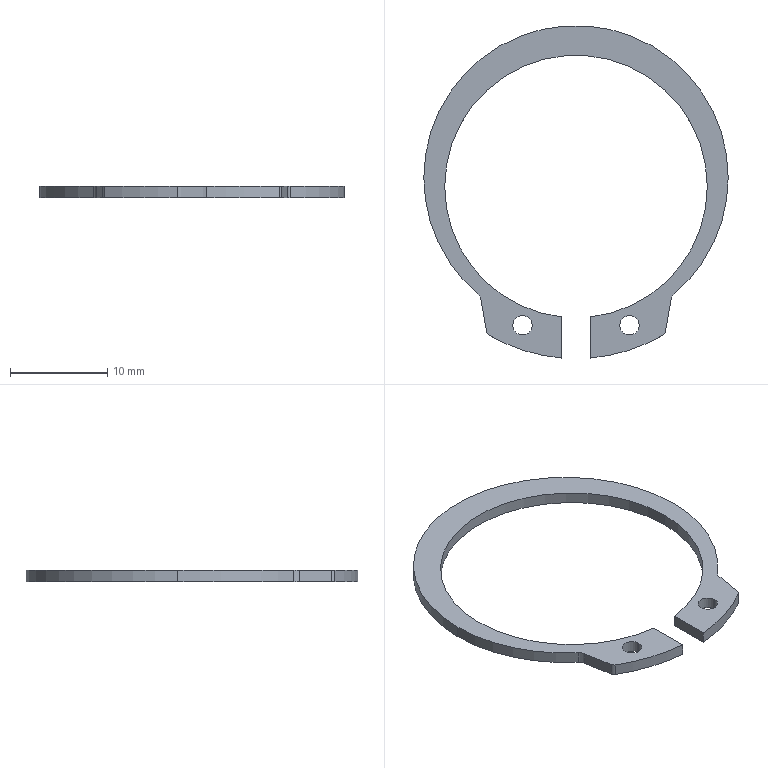Component | SolidWorks | 28mmShaftSnapRingGB896-1986-28-1 | 1 solid | 22 faces | box 31.3 x 34.19 x 1.2 mm | volume 284 mm3 | cylinder 16 | plane 6 | commonest cylinder face diameters 2 x6 31.3 x3 27 x3 1 x2 35.4 x2
STEP:
#1=CARTESIAN_POINT('',(-18.936,-4.841,97.87));
#2=VERTEX_POINT('',#1);
#3=CARTESIAN_POINT('',(-20.168,-4.841,97.87));
#4=VERTEX_POINT('',#3);
#5=CARTESIAN_POINT('',(-19.552,-4.841,97.87));
#6=DIRECTION('',(0.,0.,1.));
#7=DIRECTION('',(1.,0.,0.));
#8=AXIS2_PLACEMENT_3D('',#5,#6,#7);
#9=CIRCLE('',#8,0.6161);
#10=EDGE_CURVE('',#2,#4,#9,.T.);
#11=ORIENTED_EDGE('',*,*,#10,.T.);
#12=CARTESIAN_POINT('',(-20.168,-4.841,97.917));
#13=VERTEX_POINT('',#12);
#14=CARTESIAN_POINT('',(-20.168,-4.841,97.87));
#15=DIRECTION('',(0.,0.,1.));
#16=VECTOR('',#15,39.37);
#17=LINE('',#14,#16);
#18=EDGE_CURVE('',#4,#13,#17,.T.);
#19=ORIENTED_EDGE('',*,*,#18,.T.);
#20=CARTESIAN_POINT('',(-18.936,-4.841,97.917));
#21=VERTEX_POINT('',#20);
#22=CARTESIAN_POINT('',(-19.552,-4.841,97.917));
#23=DIRECTION('',(0.,0.,-1.));
#24=DIRECTION('',(1.,0.,0.));
#25=AXIS2_PLACEMENT_3D('',#22,#23,#24);
#26=CIRCLE('',#25,0.6161);
#27=EDGE_CURVE('',#13,#21,#26,.T.);
#28=ORIENTED_EDGE('',*,*,#27,.T.);
#29=CARTESIAN_POINT('',(-18.936,-4.841,97.87));
#30=DIRECTION('',(0.,0.,1.));
#31=VECTOR('',#30,39.37);
#32=LINE('',#29,#31);
#33=EDGE_CURVE('',#2,#21,#32,.T.);
#34=ORIENTED_EDGE('',*,*,#33,.F.);
#35=EDGE_LOOP('',(#11,#19,#28,#34));
#36=FACE_OUTER_BOUND('',#35,.T.);
#37=CARTESIAN_POINT('',(-19.552,-4.841,97.87));
#38=DIRECTION('',(0.,0.,1.));
#39=DIRECTION('',(1.,0.,0.));
#40=AXIS2_PLACEMENT_3D('',#37,#38,#39);
#41=CYLINDRICAL_SURFACE('',#40,0.6161);
#42=ADVANCED_FACE('',(#36),#41,.T.);
#43=CARTESIAN_POINT('',(-19.153,-5.312,97.87));
#44=VERTEX_POINT('',#43);
#45=CARTESIAN_POINT('',(-19.552,-4.841,97.87));
#46=DIRECTION('',(0.,0.,1.));
#47=DIRECTION('',(1.,0.,0.));
#48=AXIS2_PLACEMENT_3D('',#45,#46,#47);
#49=CIRCLE('',#48,0.6161);
#50=EDGE_CURVE('',#44,#2,#49,.T.);
#51=ORIENTED_EDGE('',*,*,#50,.T.);
#52=ORIENTED_EDGE('',*,*,#33,.T.);
#53=CARTESIAN_POINT('',(-19.153,-5.312,97.917));
#54=VERTEX_POINT('',#53);
#55=CARTESIAN_POINT('',(-19.552,-4.841,97.917));
#56=DIRECTION('',(0.,0.,-1.));
#57=DIRECTION('',(1.,0.,0.));
#58=AXIS2_PLACEMENT_3D('',#55,#56,#57);
#59=CIRCLE('',#58,0.6161);
#60=EDGE_CURVE('',#21,#54,#59,.T.);
#61=ORIENTED_EDGE('',*,*,#60,.T.);
#62=CARTESIAN_POINT('',(-19.153,-5.312,97.87));
#63=DIRECTION('',(0.,0.,-1.));
#64=VECTOR('',#63,39.37);
#65=LINE('',#62,#64);
#66=EDGE_CURVE('',#54,#44,#65,.T.);
#67=ORIENTED_EDGE('',*,*,#66,.T.);
#68=EDGE_LOOP('',(#51,#52,#61,#67));
#69=FACE_OUTER_BOUND('',#68,.T.);
#70=CARTESIAN_POINT('',(-19.552,-4.841,97.87));
#71=DIRECTION('',(0.,0.,1.));
#72=DIRECTION('',(1.,0.,0.));
#73=AXIS2_PLACEMENT_3D('',#70,#71,#72);
#74=CYLINDRICAL_SURFACE('',#73,0.6161);
#75=ADVANCED_FACE('',(#69),#74,.T.);
#76=CARTESIAN_POINT('',(-20.083,-4.877,97.87));
#77=VERTEX_POINT('',#76);
#78=CARTESIAN_POINT('',(-19.611,-5.405,97.87));
#79=VERTEX_POINT('',#78);
#80=CARTESIAN_POINT('',(-19.552,-4.877,97.87));
#81=DIRECTION('',(0.,0.,1.));
#82=DIRECTION('',(-1.,0.,0.));
#83=AXIS2_PLACEMENT_3D('',#80,#81,#82);
#84=CIRCLE('',#83,0.5315);
#85=EDGE_CURVE('',#77,#79,#84,.T.);
#86=ORIENTED_EDGE('',*,*,#85,.F.);
#87=CARTESIAN_POINT('',(-20.083,-4.877,97.917));
#88=VERTEX_POINT('',#87);
#89=CARTESIAN_POINT('',(-20.083,-4.877,97.87));
#90=DIRECTION('',(0.,0.,1.));
#91=VECTOR('',#90,39.37);
#92=LINE('',#89,#91);
#93=EDGE_CURVE('',#77,#88,#92,.T.);
#94=ORIENTED_EDGE('',*,*,#93,.T.);
#95=CARTESIAN_POINT('',(-19.611,-5.405,97.917));
#96=VERTEX_POINT('',#95);
#97=CARTESIAN_POINT('',(-19.552,-4.877,97.917));
#98=DIRECTION('',(0.,0.,1.));
#99=DIRECTION('',(-1.,0.,0.));
#100=AXIS2_PLACEMENT_3D('',#97,#98,#99);
#101=CIRCLE('',#100,0.5315);
#102=EDGE_CURVE('',#88,#96,#101,.T.);
#103=ORIENTED_EDGE('',*,*,#102,.T.);
#104=CARTESIAN_POINT('',(-19.611,-5.405,97.87));
#105=DIRECTION('',(0.,0.,1.));
#106=VECTOR('',#105,39.37);
#107=LINE('',#104,#106);
#108=EDGE_CURVE('',#79,#96,#107,.T.);
#109=ORIENTED_EDGE('',*,*,#108,.F.);
#110=EDGE_LOOP('',(#86,#94,#103,#109));
#111=FACE_OUTER_BOUND('',#110,.T.);
#112=CARTESIAN_POINT('',(-19.552,-4.877,97.87));
#113=DIRECTION('',(0.,0.,1.));
#114=DIRECTION('',(1.,0.,0.));
#115=AXIS2_PLACEMENT_3D('',#112,#113,#114);
#116=CYLINDRICAL_SURFACE('',#115,0.5315);
#117=ADVANCED_FACE('',(#111),#116,.F.);
#118=ORIENTED_EDGE('',*,*,#93,.F.);
#119=CARTESIAN_POINT('',(-19.02,-4.877,97.87));
#120=VERTEX_POINT('',#119);
#121=CARTESIAN_POINT('',(-19.552,-4.877,97.87));
#122=DIRECTION('',(0.,0.,1.));
#123=DIRECTION('',(-1.,0.,0.));
#124=AXIS2_PLACEMENT_3D('',#121,#122,#123);
#125=CIRCLE('',#124,0.5315);
#126=EDGE_CURVE('',#120,#77,#125,.T.);
#127=ORIENTED_EDGE('',*,*,#126,.F.);
#128=CARTESIAN_POINT('',(-19.02,-4.877,97.917));
#129=VERTEX_POINT('',#128);
#130=CARTESIAN_POINT('',(-19.02,-4.877,97.87));
#131=DIRECTION('',(0.,0.,1.));
#132=VECTOR('',#131,39.37);
#133=LINE('',#130,#132);
#134=EDGE_CURVE('',#120,#129,#133,.T.);
#135=ORIENTED_EDGE('',*,*,#134,.T.);
#136=CARTESIAN_POINT('',(-19.552,-4.877,97.917));
#137=DIRECTION('',(0.,0.,1.));
#138=DIRECTION('',(-1.,0.,0.));
#139=AXIS2_PLACEMENT_3D('',#136,#137,#138);
#140=CIRCLE('',#139,0.5315);
#141=EDGE_CURVE('',#129,#88,#140,.T.);
#142=ORIENTED_EDGE('',*,*,#141,.T.);
#143=EDGE_LOOP('',(#118,#127,#135,#142));
#144=FACE_OUTER_BOUND('',#143,.T.);
#145=CARTESIAN_POINT('',(-19.552,-4.877,97.87));
#146=DIRECTION('',(0.,0.,1.));
#147=DIRECTION('',(1.,0.,0.));
#148=AXIS2_PLACEMENT_3D('',#145,#146,#147);
#149=CYLINDRICAL_SURFACE('',#148,0.5315);
#150=ADVANCED_FACE('',(#144),#149,.F.);
#151=CARTESIAN_POINT('',(-19.808,-5.439,97.87));
#152=VERTEX_POINT('',#151);
#153=CARTESIAN_POINT('',(-19.729,-5.439,97.87));
#154=VERTEX_POINT('',#153);
#155=CARTESIAN_POINT('',(-19.768,-5.439,97.87));
#156=DIRECTION('',(0.,0.,1.));
#157=DIRECTION('',(1.,0.,0.));
#158=AXIS2_PLACEMENT_3D('',#155,#156,#157);
#159=CIRCLE('',#158,0.03937);
#160=EDGE_CURVE('',#152,#154,#159,.T.);
#161=ORIENTED_EDGE('',*,*,#160,.F.);
#162=CARTESIAN_POINT('',(-19.808,-5.439,97.917));
#163=VERTEX_POINT('',#162);
#164=CARTESIAN_POINT('',(-19.808,-5.439,97.87));
#165=DIRECTION('',(0.,0.,1.));
#166=VECTOR('',#165,39.37);
#167=LINE('',#164,#166);
#168=EDGE_CURVE('',#152,#163,#167,.T.);
#169=ORIENTED_EDGE('',*,*,#168,.T.);
#170=CARTESIAN_POINT('',(-19.729,-5.439,97.917));
#171=VERTEX_POINT('',#170);
#172=CARTESIAN_POINT('',(-19.768,-5.439,97.917));
#173=DIRECTION('',(0.,0.,1.));
#174=DIRECTION('',(1.,0.,0.));
#175=AXIS2_PLACEMENT_3D('',#172,#173,#174);
#176=CIRCLE('',#175,0.03937);
#177=EDGE_CURVE('',#163,#171,#176,.T.);
#178=ORIENTED_EDGE('',*,*,#177,.T.);
#179=CARTESIAN_POINT('',(-19.729,-5.439,97.87));
#180=DIRECTION('',(0.,0.,1.));
#181=VECTOR('',#180,39.37);
#182=LINE('',#179,#181);
#183=EDGE_CURVE('',#154,#171,#182,.T.);
#184=ORIENTED_EDGE('',*,*,#183,.F.);
#185=EDGE_LOOP('',(#161,#169,#178,#184));
#186=FACE_OUTER_BOUND('',#185,.T.);
#187=CARTESIAN_POINT('',(-19.768,-5.439,97.87));
#188=DIRECTION('',(0.,0.,1.));
#189=DIRECTION('',(1.,0.,0.));
#190=AXIS2_PLACEMENT_3D('',#187,#188,#189);
#191=CYLINDRICAL_SURFACE('',#190,0.03937);
#192=ADVANCED_FACE('',(#186),#191,.F.);
#193=CARTESIAN_POINT('',(-19.374,-5.439,97.87));
#194=VERTEX_POINT('',#193);
#195=CARTESIAN_POINT('',(-19.296,-5.439,97.87));
#196=VERTEX_POINT('',#195);
#197=CARTESIAN_POINT('',(-19.335,-5.439,97.87));
#198=DIRECTION('',(0.,0.,1.));
#199=DIRECTION('',(1.,0.,0.));
#200=AXIS2_PLACEMENT_3D('',#197,#198,#199);
#201=CIRCLE('',#200,0.03937);
#202=EDGE_CURVE('',#194,#196,#201,.T.);
#203=ORIENTED_EDGE('',*,*,#202,.F.);
#204=CARTESIAN_POINT('',(-19.374,-5.439,97.917));
#205=VERTEX_POINT('',#204);
#206=CARTESIAN_POINT('',(-19.374,-5.439,97.87));
#207=DIRECTION('',(0.,0.,1.));
#208=VECTOR('',#207,39.37);
#209=LINE('',#206,#208);
#210=EDGE_CURVE('',#194,#205,#209,.T.);
#211=ORIENTED_EDGE('',*,*,#210,.T.);
#212=CARTESIAN_POINT('',(-19.296,-5.439,97.917));
#213=VERTEX_POINT('',#212);
#214=CARTESIAN_POINT('',(-19.335,-5.439,97.917));
#215=DIRECTION('',(0.,0.,1.));
#216=DIRECTION('',(1.,0.,0.));
#217=AXIS2_PLACEMENT_3D('',#214,#215,#216);
#218=CIRCLE('',#217,0.03937);
#219=EDGE_CURVE('',#205,#213,#218,.T.);
#220=ORIENTED_EDGE('',*,*,#219,.T.);
#221=CARTESIAN_POINT('',(-19.296,-5.439,97.87));
#222=DIRECTION('',(0.,0.,1.));
#223=VECTOR('',#222,39.37);
#224=LINE('',#221,#223);
#225=EDGE_CURVE('',#196,#213,#224,.T.);
#226=ORIENTED_EDGE('',*,*,#225,.F.);
#227=EDGE_LOOP('',(#203,#211,#220,#226));
#228=FACE_OUTER_BOUND('',#227,.T.);
#229=CARTESIAN_POINT('',(-19.335,-5.439,97.87));
#230=DIRECTION('',(0.,0.,1.));
#231=DIRECTION('',(1.,0.,0.));
#232=AXIS2_PLACEMENT_3D('',#229,#230,#231);
#233=CYLINDRICAL_SURFACE('',#232,0.03937);
#234=ADVANCED_FACE('',(#228),#233,.F.);
#235=CARTESIAN_POINT('',(-19.167,-5.335,97.917));
#236=VERTEX_POINT('',#235);
#237=CARTESIAN_POINT('',(-19.128,-5.342,97.917));
#238=DIRECTION('',(0.,0.,1.));
#239=DIRECTION('',(1.,0.,0.));
#240=AXIS2_PLACEMENT_3D('',#237,#238,#239);
#241=CIRCLE('',#240,0.03937);
#242=EDGE_CURVE('',#54,#236,#241,.T.);
#243=ORIENTED_EDGE('',*,*,#242,.F.);
#244=ORIENTED_EDGE('',*,*,#60,.F.);
#245=ORIENTED_EDGE('',*,*,#27,.F.);
#246=CARTESIAN_POINT('',(-19.95,-5.312,97.917));
#247=VERTEX_POINT('',#246);
#248=CARTESIAN_POINT('',(-19.552,-4.841,97.917));
#249=DIRECTION('',(0.,0.,-1.));
#250=DIRECTION('',(1.,0.,0.));
#251=AXIS2_PLACEMENT_3D('',#248,#249,#250);
#252=CIRCLE('',#251,0.6161);
#253=EDGE_CURVE('',#247,#13,#252,.T.);
#254=ORIENTED_EDGE('',*,*,#253,.F.);
#255=CARTESIAN_POINT('',(-19.937,-5.335,97.917));
#256=VERTEX_POINT('',#255);
#257=CARTESIAN_POINT('',(-19.975,-5.342,97.917));
#258=DIRECTION('',(0.,0.,1.));
#259=DIRECTION('',(1.,0.,0.));
#260=AXIS2_PLACEMENT_3D('',#257,#258,#259);
#261=CIRCLE('',#260,0.03937);
#262=EDGE_CURVE('',#256,#247,#261,.T.);
#263=ORIENTED_EDGE('',*,*,#262,.F.);
#264=CARTESIAN_POINT('',(-19.914,-5.464,97.917));
#265=VERTEX_POINT('',#264);
#266=CARTESIAN_POINT('',(-19.914,-5.464,97.917));
#267=DIRECTION('',(-0.1736,0.9848,0.));
#268=VECTOR('',#267,39.37);
#269=LINE('',#266,#268);
#270=EDGE_CURVE('',#265,#256,#269,.T.);
#271=ORIENTED_EDGE('',*,*,#270,.F.);
#272=CARTESIAN_POINT('',(-19.904,-5.478,97.917));
#273=VERTEX_POINT('',#272);
#274=CARTESIAN_POINT('',(-19.894,-5.461,97.917));
#275=DIRECTION('',(0.,0.,-1.));
#276=DIRECTION('',(1.,0.,0.));
#277=AXIS2_PLACEMENT_3D('',#274,#275,#276);
#278=CIRCLE('',#277,0.01969);
#279=EDGE_CURVE('',#273,#265,#278,.T.);
#280=ORIENTED_EDGE('',*,*,#279,.F.);
#281=CARTESIAN_POINT('',(-19.611,-5.571,97.917));
#282=VERTEX_POINT('',#281);
#283=CARTESIAN_POINT('',(-19.552,-4.877,97.917));
#284=DIRECTION('',(0.,0.,-1.));
#285=DIRECTION('',(1.,0.,0.));
#286=AXIS2_PLACEMENT_3D('',#283,#284,#285);
#287=CIRCLE('',#286,0.6969);
#288=EDGE_CURVE('',#282,#273,#287,.T.);
#289=ORIENTED_EDGE('',*,*,#288,.F.);
#290=CARTESIAN_POINT('',(-19.611,-4.877,97.917));
#291=DIRECTION('',(0.,-1.,0.));
#292=VECTOR('',#291,39.37);
#293=LINE('',#290,#292);
#294=EDGE_CURVE('',#96,#282,#293,.T.);
#295=ORIENTED_EDGE('',*,*,#294,.F.);
#296=ORIENTED_EDGE('',*,*,#102,.F.);
#297=ORIENTED_EDGE('',*,*,#141,.F.);
#298=CARTESIAN_POINT('',(-19.493,-5.405,97.917));
#299=VERTEX_POINT('',#298);
#300=CARTESIAN_POINT('',(-19.552,-4.877,97.917));
#301=DIRECTION('',(0.,0.,1.));
#302=DIRECTION('',(-1.,0.,0.));
#303=AXIS2_PLACEMENT_3D('',#300,#301,#302);
#304=CIRCLE('',#303,0.5315);
#305=EDGE_CURVE('',#299,#129,#304,.T.);
#306=ORIENTED_EDGE('',*,*,#305,.F.);
#307=CARTESIAN_POINT('',(-19.493,-5.571,97.917));
#308=VERTEX_POINT('',#307);
#309=CARTESIAN_POINT('',(-19.493,-4.877,97.917));
#310=DIRECTION('',(0.,1.,0.));
#311=VECTOR('',#310,39.37);
#312=LINE('',#309,#311);
#313=EDGE_CURVE('',#308,#299,#312,.T.);
#314=ORIENTED_EDGE('',*,*,#313,.F.);
#315=CARTESIAN_POINT('',(-19.199,-5.478,97.917));
#316=VERTEX_POINT('',#315);
#317=CARTESIAN_POINT('',(-19.552,-4.877,97.917));
#318=DIRECTION('',(0.,0.,-1.));
#319=DIRECTION('',(1.,0.,0.));
#320=AXIS2_PLACEMENT_3D('',#317,#318,#319);
#321=CIRCLE('',#320,0.6969);
#322=EDGE_CURVE('',#316,#308,#321,.T.);
#323=ORIENTED_EDGE('',*,*,#322,.F.);
#324=CARTESIAN_POINT('',(-19.19,-5.464,97.917));
#325=VERTEX_POINT('',#324);
#326=CARTESIAN_POINT('',(-19.209,-5.461,97.917));
#327=DIRECTION('',(0.,0.,-1.));
#328=DIRECTION('',(1.,0.,0.));
#329=AXIS2_PLACEMENT_3D('',#326,#327,#328);
#330=CIRCLE('',#329,0.01969);
#331=EDGE_CURVE('',#325,#316,#330,.T.);
#332=ORIENTED_EDGE('',*,*,#331,.F.);
#333=CARTESIAN_POINT('',(-19.167,-5.335,97.917));
#334=DIRECTION('',(-0.1736,-0.9848,0.));
#335=VECTOR('',#334,39.37);
#336=LINE('',#333,#335);
#337=EDGE_CURVE('',#236,#325,#336,.T.);
#338=ORIENTED_EDGE('',*,*,#337,.F.);
#339=EDGE_LOOP('',(#243,#244,#245,#254,#263,#271,#280,#289,#295,#296,#297,#306,#314,#323,#332,#338));
#340=FACE_OUTER_BOUND('',#339,.T.);
#341=CARTESIAN_POINT('',(-19.768,-5.439,97.917));
#342=DIRECTION('',(0.,0.,1.));
#343=DIRECTION('',(1.,0.,0.));
#344=AXIS2_PLACEMENT_3D('',#341,#342,#343);
#345=CIRCLE('',#344,0.03937);
#346=EDGE_CURVE('',#171,#163,#345,.T.);
#347=ORIENTED_EDGE('',*,*,#346,.F.);
#348=ORIENTED_EDGE('',*,*,#177,.F.);
#349=EDGE_LOOP('',(#347,#348));
#350=FACE_BOUND('',#349,.T.);
#351=CARTESIAN_POINT('',(-19.335,-5.439,97.917));
#352=DIRECTION('',(0.,0.,1.));
#353=DIRECTION('',(1.,0.,0.));
#354=AXIS2_PLACEMENT_3D('',#351,#352,#353);
#355=CIRCLE('',#354,0.03937);
#356=EDGE_CURVE('',#213,#205,#355,.T.);
#357=ORIENTED_EDGE('',*,*,#356,.F.);
#358=ORIENTED_EDGE('',*,*,#219,.F.);
#359=EDGE_LOOP('',(#357,#358));
#360=FACE_BOUND('',#359,.T.);
#361=CARTESIAN_POINT('',(-19.552,-4.877,97.917));
#362=DIRECTION('',(0.,0.,-1.));
#363=DIRECTION('',(-1.,0.,0.));
#364=AXIS2_PLACEMENT_3D('',#361,#362,#363);
#365=PLANE('',#364);
#366=ADVANCED_FACE('',(#340,#350,#360),#365,.F.);
#367=ORIENTED_EDGE('',*,*,#18,.F.);
#368=CARTESIAN_POINT('',(-19.95,-5.312,97.87));
#369=VERTEX_POINT('',#368);
#370=CARTESIAN_POINT('',(-19.552,-4.841,97.87));
#371=DIRECTION('',(0.,0.,1.));
#372=DIRECTION('',(1.,0.,0.));
#373=AXIS2_PLACEMENT_3D('',#370,#371,#372);
#374=CIRCLE('',#373,0.6161);
#375=EDGE_CURVE('',#4,#369,#374,.T.);
#376=ORIENTED_EDGE('',*,*,#375,.T.);
#377=CARTESIAN_POINT('',(-19.95,-5.312,97.87));
#378=DIRECTION('',(0.,0.,1.));
#379=VECTOR('',#378,39.37);
#380=LINE('',#377,#379);
#381=EDGE_CURVE('',#369,#247,#380,.T.);
#382=ORIENTED_EDGE('',*,*,#381,.T.);
#383=ORIENTED_EDGE('',*,*,#253,.T.);
#384=EDGE_LOOP('',(#367,#376,#382,#383));
#385=FACE_OUTER_BOUND('',#384,.T.);
#386=CARTESIAN_POINT('',(-19.552,-4.841,97.87));
#387=DIRECTION('',(0.,0.,1.));
#388=DIRECTION('',(1.,0.,0.));
#389=AXIS2_PLACEMENT_3D('',#386,#387,#388);
#390=CYLINDRICAL_SURFACE('',#389,0.6161);
#391=ADVANCED_FACE('',(#385),#390,.T.);
#392=CARTESIAN_POINT('',(-19.937,-5.335,97.87));
#393=VERTEX_POINT('',#392);
#394=CARTESIAN_POINT('',(-19.937,-5.335,97.87));
#395=DIRECTION('',(0.,0.,-1.));
#396=VECTOR('',#395,39.37);
#397=LINE('',#394,#396);
#398=EDGE_CURVE('',#256,#393,#397,.T.);
#399=ORIENTED_EDGE('',*,*,#398,.F.);
#400=ORIENTED_EDGE('',*,*,#262,.T.);
#401=ORIENTED_EDGE('',*,*,#381,.F.);
#402=CARTESIAN_POINT('',(-19.975,-5.342,97.87));
#403=DIRECTION('',(0.,0.,1.));
#404=DIRECTION('',(1.,0.,0.));
#405=AXIS2_PLACEMENT_3D('',#402,#403,#404);
#406=CIRCLE('',#405,0.03937);
#407=EDGE_CURVE('',#393,#369,#406,.T.);
#408=ORIENTED_EDGE('',*,*,#407,.F.);
#409=EDGE_LOOP('',(#399,#400,#401,#408));
#410=FACE_OUTER_BOUND('',#409,.T.);
#411=CARTESIAN_POINT('',(-19.975,-5.342,97.87));
#412=DIRECTION('',(0.,0.,1.));
#413=DIRECTION('',(1.,0.,0.));
#414=AXIS2_PLACEMENT_3D('',#411,#412,#413);
#415=CYLINDRICAL_SURFACE('',#414,0.03937);
#416=ADVANCED_FACE('',(#410),#415,.F.);
#417=CARTESIAN_POINT('',(-19.914,-5.464,97.87));
#418=VERTEX_POINT('',#417);
#419=CARTESIAN_POINT('',(-19.939,-5.321,97.87));
#420=DIRECTION('',(0.1736,-0.9848,0.));
#421=VECTOR('',#420,39.37);
#422=LINE('',#419,#421);
#423=EDGE_CURVE('',#393,#418,#422,.T.);
#424=ORIENTED_EDGE('',*,*,#423,.T.);
#425=CARTESIAN_POINT('',(-19.914,-5.464,97.87));
#426=DIRECTION('',(0.,0.,1.));
#427=VECTOR('',#426,39.37);
#428=LINE('',#425,#427);
#429=EDGE_CURVE('',#418,#265,#428,.T.);
#430=ORIENTED_EDGE('',*,*,#429,.T.);
#431=ORIENTED_EDGE('',*,*,#270,.T.);
#432=ORIENTED_EDGE('',*,*,#398,.T.);
#433=EDGE_LOOP('',(#424,#430,#431,#432));
#434=FACE_OUTER_BOUND('',#433,.T.);
#435=CARTESIAN_POINT('',(-19.939,-5.321,97.87));
#436=DIRECTION('',(-0.9848,-0.1736,0.));
#437=DIRECTION('',(0.1736,-0.9848,0.));
#438=AXIS2_PLACEMENT_3D('',#435,#436,#437);
#439=PLANE('',#438);
#440=ADVANCED_FACE('',(#434),#439,.T.);
#441=ORIENTED_EDGE('',*,*,#279,.T.);
#442=ORIENTED_EDGE('',*,*,#429,.F.);
#443=CARTESIAN_POINT('',(-19.904,-5.478,97.87));
#444=VERTEX_POINT('',#443);
#445=CARTESIAN_POINT('',(-19.894,-5.461,97.87));
#446=DIRECTION('',(0.,0.,1.));
#447=DIRECTION('',(1.,0.,0.));
#448=AXIS2_PLACEMENT_3D('',#445,#446,#447);
#449=CIRCLE('',#448,0.01969);
#450=EDGE_CURVE('',#418,#444,#449,.T.);
#451=ORIENTED_EDGE('',*,*,#450,.T.);
#452=CARTESIAN_POINT('',(-19.904,-5.478,97.87));
#453=DIRECTION('',(0.,0.,1.));
#454=VECTOR('',#453,39.37);
#455=LINE('',#452,#454);
#456=EDGE_CURVE('',#444,#273,#455,.T.);
#457=ORIENTED_EDGE('',*,*,#456,.T.);
#458=EDGE_LOOP('',(#441,#442,#451,#457));
#459=FACE_OUTER_BOUND('',#458,.T.);
#460=CARTESIAN_POINT('',(-19.894,-5.461,97.87));
#461=DIRECTION('',(0.,0.,1.));
#462=DIRECTION('',(1.,0.,0.));
#463=AXIS2_PLACEMENT_3D('',#460,#461,#462);
#464=CYLINDRICAL_SURFACE('',#463,0.01969);
#465=ADVANCED_FACE('',(#459),#464,.T.);
#466=CARTESIAN_POINT('',(-19.611,-5.571,97.87));
#467=VERTEX_POINT('',#466);
#468=CARTESIAN_POINT('',(-19.552,-4.877,97.87));
#469=DIRECTION('',(0.,0.,1.));
#470=DIRECTION('',(1.,0.,0.));
#471=AXIS2_PLACEMENT_3D('',#468,#469,#470);
#472=CIRCLE('',#471,0.6969);
#473=EDGE_CURVE('',#444,#467,#472,.T.);
#474=ORIENTED_EDGE('',*,*,#473,.T.);
#475=CARTESIAN_POINT('',(-19.611,-5.571,97.87));
#476=DIRECTION('',(0.,0.,1.));
#477=VECTOR('',#476,39.37);
#478=LINE('',#475,#477);
#479=EDGE_CURVE('',#467,#282,#478,.T.);
#480=ORIENTED_EDGE('',*,*,#479,.T.);
#481=ORIENTED_EDGE('',*,*,#288,.T.);
#482=ORIENTED_EDGE('',*,*,#456,.F.);
#483=EDGE_LOOP('',(#474,#480,#481,#482));
#484=FACE_OUTER_BOUND('',#483,.T.);
#485=CARTESIAN_POINT('',(-19.552,-4.877,97.87));
#486=DIRECTION('',(0.,0.,1.));
#487=DIRECTION('',(1.,0.,0.));
#488=AXIS2_PLACEMENT_3D('',#485,#486,#487);
#489=CYLINDRICAL_SURFACE('',#488,0.6969);
#490=ADVANCED_FACE('',(#484),#489,.T.);
#491=CARTESIAN_POINT('',(-19.611,-5.383,97.87));
#492=DIRECTION('',(0.,1.,0.));
#493=VECTOR('',#492,39.37);
#494=LINE('',#491,#493);
#495=EDGE_CURVE('',#467,#79,#494,.T.);
#496=ORIENTED_EDGE('',*,*,#495,.T.);
#497=ORIENTED_EDGE('',*,*,#108,.T.);
#498=ORIENTED_EDGE('',*,*,#294,.T.);
#499=ORIENTED_EDGE('',*,*,#479,.F.);
#500=EDGE_LOOP('',(#496,#497,#498,#499));
#501=FACE_OUTER_BOUND('',#500,.T.);
#502=CARTESIAN_POINT('',(-19.611,-5.383,97.87));
#503=DIRECTION('',(1.,0.,0.));
#504=DIRECTION('',(0.,0.,-1.));
#505=AXIS2_PLACEMENT_3D('',#502,#503,#504);
#506=PLANE('',#505);
#507=ADVANCED_FACE('',(#501),#506,.T.);
#508=ORIENTED_EDGE('',*,*,#134,.F.);
#509=CARTESIAN_POINT('',(-19.493,-5.405,97.87));
#510=VERTEX_POINT('',#509);
#511=CARTESIAN_POINT('',(-19.552,-4.877,97.87));
#512=DIRECTION('',(0.,0.,1.));
#513=DIRECTION('',(-1.,0.,0.));
#514=AXIS2_PLACEMENT_3D('',#511,#512,#513);
#515=CIRCLE('',#514,0.5315);
#516=EDGE_CURVE('',#510,#120,#515,.T.);
#517=ORIENTED_EDGE('',*,*,#516,.F.);
#518=CARTESIAN_POINT('',(-19.493,-5.405,97.917));
#519=DIRECTION('',(0.,0.,-1.));
#520=VECTOR('',#519,39.37);
#521=LINE('',#518,#520);
#522=EDGE_CURVE('',#299,#510,#521,.T.);
#523=ORIENTED_EDGE('',*,*,#522,.F.);
#524=ORIENTED_EDGE('',*,*,#305,.T.);
#525=EDGE_LOOP('',(#508,#517,#523,#524));
#526=FACE_OUTER_BOUND('',#525,.T.);
#527=CARTESIAN_POINT('',(-19.552,-4.877,97.87));
#528=DIRECTION('',(0.,0.,1.));
#529=DIRECTION('',(1.,0.,0.));
#530=AXIS2_PLACEMENT_3D('',#527,#528,#529);
#531=CYLINDRICAL_SURFACE('',#530,0.5315);
#532=ADVANCED_FACE('',(#526),#531,.F.);
#533=CARTESIAN_POINT('',(-19.493,-5.571,97.87));
#534=VERTEX_POINT('',#533);
#535=CARTESIAN_POINT('',(-19.493,-5.383,97.87));
#536=DIRECTION('',(0.,-1.,0.));
#537=VECTOR('',#536,39.37);
#538=LINE('',#535,#537);
#539=EDGE_CURVE('',#510,#534,#538,.T.);
#540=ORIENTED_EDGE('',*,*,#539,.T.);
#541=CARTESIAN_POINT('',(-19.493,-5.571,97.87));
#542=DIRECTION('',(0.,0.,1.));
#543=VECTOR('',#542,39.37);
#544=LINE('',#541,#543);
#545=EDGE_CURVE('',#534,#308,#544,.T.);
#546=ORIENTED_EDGE('',*,*,#545,.T.);
#547=ORIENTED_EDGE('',*,*,#313,.T.);
#548=ORIENTED_EDGE('',*,*,#522,.T.);
#549=EDGE_LOOP('',(#540,#546,#547,#548));
#550=FACE_OUTER_BOUND('',#549,.T.);
#551=CARTESIAN_POINT('',(-19.493,-5.383,97.87));
#552=DIRECTION('',(-1.,0.,0.));
#553=DIRECTION('',(0.,0.,1.));
#554=AXIS2_PLACEMENT_3D('',#551,#552,#553);
#555=PLANE('',#554);
#556=ADVANCED_FACE('',(#550),#555,.T.);
#557=ORIENTED_EDGE('',*,*,#322,.T.);
#558=ORIENTED_EDGE('',*,*,#545,.F.);
#559=CARTESIAN_POINT('',(-19.199,-5.478,97.87));
#560=VERTEX_POINT('',#559);
#561=CARTESIAN_POINT('',(-19.552,-4.877,97.87));
#562=DIRECTION('',(0.,0.,1.));
#563=DIRECTION('',(1.,0.,0.));
#564=AXIS2_PLACEMENT_3D('',#561,#562,#563);
#565=CIRCLE('',#564,0.6969);
#566=EDGE_CURVE('',#534,#560,#565,.T.);
#567=ORIENTED_EDGE('',*,*,#566,.T.);
#568=CARTESIAN_POINT('',(-19.199,-5.478,97.87));
#569=DIRECTION('',(0.,0.,1.));
#570=VECTOR('',#569,39.37);
#571=LINE('',#568,#570);
#572=EDGE_CURVE('',#560,#316,#571,.T.);
#573=ORIENTED_EDGE('',*,*,#572,.T.);
#574=EDGE_LOOP('',(#557,#558,#567,#573));
#575=FACE_OUTER_BOUND('',#574,.T.);
#576=CARTESIAN_POINT('',(-19.552,-4.877,97.87));
#577=DIRECTION('',(0.,0.,1.));
#578=DIRECTION('',(1.,0.,0.));
#579=AXIS2_PLACEMENT_3D('',#576,#577,#578);
#580=CYLINDRICAL_SURFACE('',#579,0.6969);
#581=ADVANCED_FACE('',(#575),#580,.T.);
#582=ORIENTED_EDGE('',*,*,#331,.T.);
#583=ORIENTED_EDGE('',*,*,#572,.F.);
#584=CARTESIAN_POINT('',(-19.19,-5.464,97.87));
#585=VERTEX_POINT('',#584);
#586=CARTESIAN_POINT('',(-19.209,-5.461,97.87));
#587=DIRECTION('',(0.,0.,1.));
#588=DIRECTION('',(1.,0.,0.));
#589=AXIS2_PLACEMENT_3D('',#586,#587,#588);
#590=CIRCLE('',#589,0.01969);
#591=EDGE_CURVE('',#560,#585,#590,.T.);
#592=ORIENTED_EDGE('',*,*,#591,.T.);
#593=CARTESIAN_POINT('',(-19.19,-5.464,97.87));
#594=DIRECTION('',(0.,0.,1.));
#595=VECTOR('',#594,39.37);
#596=LINE('',#593,#595);
#597=EDGE_CURVE('',#585,#325,#596,.T.);
#598=ORIENTED_EDGE('',*,*,#597,.T.);
#599=EDGE_LOOP('',(#582,#583,#592,#598));
#600=FACE_OUTER_BOUND('',#599,.T.);
#601=CARTESIAN_POINT('',(-19.209,-5.461,97.87));
#602=DIRECTION('',(0.,0.,1.));
#603=DIRECTION('',(1.,0.,0.));
#604=AXIS2_PLACEMENT_3D('',#601,#602,#603);
#605=CYLINDRICAL_SURFACE('',#604,0.01969);
#606=ADVANCED_FACE('',(#600),#605,.T.);
#607=ORIENTED_EDGE('',*,*,#337,.T.);
#608=ORIENTED_EDGE('',*,*,#597,.F.);
#609=CARTESIAN_POINT('',(-19.167,-5.335,97.87));
#610=VERTEX_POINT('',#609);
#611=CARTESIAN_POINT('',(-19.164,-5.321,97.87));
#612=DIRECTION('',(0.1736,0.9848,0.));
#613=VECTOR('',#612,39.37);
#614=LINE('',#611,#613);
#615=EDGE_CURVE('',#585,#610,#614,.T.);
#616=ORIENTED_EDGE('',*,*,#615,.T.);
#617=CARTESIAN_POINT('',(-19.167,-5.335,97.87));
#618=DIRECTION('',(0.,0.,1.));
#619=VECTOR('',#618,39.37);
#620=LINE('',#617,#619);
#621=EDGE_CURVE('',#610,#236,#620,.T.);
#622=ORIENTED_EDGE('',*,*,#621,.T.);
#623=EDGE_LOOP('',(#607,#608,#616,#622));
#624=FACE_OUTER_BOUND('',#623,.T.);
#625=CARTESIAN_POINT('',(-19.164,-5.321,97.87));
#626=DIRECTION('',(0.9848,-0.1736,0.));
#627=DIRECTION('',(0.1736,0.9848,0.));
#628=AXIS2_PLACEMENT_3D('',#625,#626,#627);
#629=PLANE('',#628);
#630=ADVANCED_FACE('',(#624),#629,.T.);
#631=ORIENTED_EDGE('',*,*,#66,.F.);
#632=ORIENTED_EDGE('',*,*,#242,.T.);
#633=ORIENTED_EDGE('',*,*,#621,.F.);
#634=CARTESIAN_POINT('',(-19.128,-5.342,97.87));
#635=DIRECTION('',(0.,0.,1.));
#636=DIRECTION('',(1.,0.,0.));
#637=AXIS2_PLACEMENT_3D('',#634,#635,#636);
#638=CIRCLE('',#637,0.03937);
#639=EDGE_CURVE('',#44,#610,#638,.T.);
#640=ORIENTED_EDGE('',*,*,#639,.F.);
#641=EDGE_LOOP('',(#631,#632,#633,#640));
#642=FACE_OUTER_BOUND('',#641,.T.);
#643=CARTESIAN_POINT('',(-19.128,-5.342,97.87));
#644=DIRECTION('',(0.,0.,1.));
#645=DIRECTION('',(1.,0.,0.));
#646=AXIS2_PLACEMENT_3D('',#643,#644,#645);
#647=CYLINDRICAL_SURFACE('',#646,0.03937);
#648=ADVANCED_FACE('',(#642),#647,.F.);
#649=ORIENTED_EDGE('',*,*,#168,.F.);
#650=CARTESIAN_POINT('',(-19.768,-5.439,97.87));
#651=DIRECTION('',(0.,0.,1.));
#652=DIRECTION('',(1.,0.,0.));
#653=AXIS2_PLACEMENT_3D('',#650,#651,#652);
#654=CIRCLE('',#653,0.03937);
#655=EDGE_CURVE('',#154,#152,#654,.T.);
#656=ORIENTED_EDGE('',*,*,#655,.F.);
#657=ORIENTED_EDGE('',*,*,#183,.T.);
#658=ORIENTED_EDGE('',*,*,#346,.T.);
#659=EDGE_LOOP('',(#649,#656,#657,#658));
#660=FACE_OUTER_BOUND('',#659,.T.);
#661=CARTESIAN_POINT('',(-19.768,-5.439,97.87));
#662=DIRECTION('',(0.,0.,1.));
#663=DIRECTION('',(1.,0.,0.));
#664=AXIS2_PLACEMENT_3D('',#661,#662,#663);
#665=CYLINDRICAL_SURFACE('',#664,0.03937);
#666=ADVANCED_FACE('',(#660),#665,.F.);
#667=ORIENTED_EDGE('',*,*,#210,.F.);
#668=CARTESIAN_POINT('',(-19.335,-5.439,97.87));
#669=DIRECTION('',(0.,0.,1.));
#670=DIRECTION('',(1.,0.,0.));
#671=AXIS2_PLACEMENT_3D('',#668,#669,#670);
#672=CIRCLE('',#671,0.03937);
#673=EDGE_CURVE('',#196,#194,#672,.T.);
#674=ORIENTED_EDGE('',*,*,#673,.F.);
#675=ORIENTED_EDGE('',*,*,#225,.T.);
#676=ORIENTED_EDGE('',*,*,#356,.T.);
#677=EDGE_LOOP('',(#667,#674,#675,#676));
#678=FACE_OUTER_BOUND('',#677,.T.);
#679=CARTESIAN_POINT('',(-19.335,-5.439,97.87));
#680=DIRECTION('',(0.,0.,1.));
#681=DIRECTION('',(1.,0.,0.));
#682=AXIS2_PLACEMENT_3D('',#679,#680,#681);
#683=CYLINDRICAL_SURFACE('',#682,0.03937);
#684=ADVANCED_FACE('',(#678),#683,.F.);
#685=ORIENTED_EDGE('',*,*,#516,.T.);
#686=ORIENTED_EDGE('',*,*,#126,.T.);
#687=ORIENTED_EDGE('',*,*,#85,.T.);
#688=ORIENTED_EDGE('',*,*,#495,.F.);
#689=ORIENTED_EDGE('',*,*,#473,.F.);
#690=ORIENTED_EDGE('',*,*,#450,.F.);
#691=ORIENTED_EDGE('',*,*,#423,.F.);
#692=ORIENTED_EDGE('',*,*,#407,.T.);
#693=ORIENTED_EDGE('',*,*,#375,.F.);
#694=ORIENTED_EDGE('',*,*,#10,.F.);
#695=ORIENTED_EDGE('',*,*,#50,.F.);
#696=ORIENTED_EDGE('',*,*,#639,.T.);
#697=ORIENTED_EDGE('',*,*,#615,.F.);
#698=ORIENTED_EDGE('',*,*,#591,.F.);
#699=ORIENTED_EDGE('',*,*,#566,.F.);
#700=ORIENTED_EDGE('',*,*,#539,.F.);
#701=EDGE_LOOP('',(#685,#686,#687,#688,#689,#690,#691,#692,#693,#694,#695,#696,#697,#698,#699,#700));
#702=FACE_OUTER_BOUND('',#701,.T.);
#703=ORIENTED_EDGE('',*,*,#655,.T.);
#704=ORIENTED_EDGE('',*,*,#160,.T.);
#705=EDGE_LOOP('',(#703,#704));
#706=FACE_BOUND('',#705,.T.);
#707=ORIENTED_EDGE('',*,*,#673,.T.);
#708=ORIENTED_EDGE('',*,*,#202,.T.);
#709=EDGE_LOOP('',(#707,#708));
#710=FACE_BOUND('',#709,.T.);
#711=CARTESIAN_POINT('',(-19.552,-4.877,97.87));
#712=DIRECTION('',(0.,0.,-1.));
#713=DIRECTION('',(-1.,0.,0.));
#714=AXIS2_PLACEMENT_3D('',#711,#712,#713);
#715=PLANE('',#714);
#716=ADVANCED_FACE('',(#702,#706,#710),#715,.T.);
#717=CLOSED_SHELL('',(#42,#75,#117,#150,#192,#234,#366,#391,#416,#440,#465,#490,#507,#532,#556,#581,#606,#630,#648,#666,#684,#716));
#718=MANIFOLD_SOLID_BREP('',#717);
#719=CARTESIAN_POINT('',(0.,0.,0.));
#720=DIRECTION('',(0.,0.,1.));
#721=DIRECTION('',(1.,0.,0.));
#722=AXIS2_PLACEMENT_3D('',#719,#720,#721);
#723=(LENGTH_UNIT()NAMED_UNIT(*)SI_UNIT($,.METRE.));
#724=LENGTH_MEASURE_WITH_UNIT(LENGTH_MEASURE(0.0254),#723);
#725=DIMENSIONAL_EXPONENTS(1.,0.,0.,0.,0.,0.,0.);
#726=(CONVERSION_BASED_UNIT('',#724)LENGTH_UNIT()NAMED_UNIT(#725));
#727=UNCERTAINTY_MEASURE_WITH_UNIT(LENGTH_MEASURE(0.00001),#726,'','');
#728=(NAMED_UNIT(*)PLANE_ANGLE_UNIT()SI_UNIT($,.RADIAN.));
#729=(NAMED_UNIT(*)SI_UNIT($,.STERADIAN.)SOLID_ANGLE_UNIT());
#730=(GEOMETRIC_REPRESENTATION_CONTEXT(3)GLOBAL_UNCERTAINTY_ASSIGNED_CONTEXT((#727))GLOBAL_UNIT_ASSIGNED_CONTEXT((#726,#728,#729))REPRESENTATION_CONTEXT('',''));
#731=ADVANCED_BREP_SHAPE_REPRESENTATION('',(#718,#722),#730);
#732=COLOUR_RGB('',0.7922,0.8196,0.9333);
#733=FILL_AREA_STYLE_COLOUR('',#732);
#734=FILL_AREA_STYLE('',(#733));
#735=SURFACE_STYLE_FILL_AREA(#734);
#736=SURFACE_SIDE_STYLE('',(#735));
#737=SURFACE_STYLE_USAGE(.BOTH.,#736);
#738=PRESENTATION_STYLE_ASSIGNMENT((#737));
#739=STYLED_ITEM('',(#738),#718);
#740=PRESENTATION_LAYER_ASSIGNMENT('','',(#739));
#741=(LENGTH_UNIT()NAMED_UNIT(*)SI_UNIT($,.METRE.));
#742=LENGTH_MEASURE_WITH_UNIT(LENGTH_MEASURE(0.0254),#741);
#743=DIMENSIONAL_EXPONENTS(1.,0.,0.,0.,0.,0.,0.);
#744=(CONVERSION_BASED_UNIT('',#742)LENGTH_UNIT()NAMED_UNIT(#743));
#745=UNCERTAINTY_MEASURE_WITH_UNIT(LENGTH_MEASURE(0.00001),#744,'','');
#746=(NAMED_UNIT(*)PLANE_ANGLE_UNIT()SI_UNIT($,.RADIAN.));
#747=(NAMED_UNIT(*)SI_UNIT($,.STERADIAN.)SOLID_ANGLE_UNIT());
#748=(GEOMETRIC_REPRESENTATION_CONTEXT(3)GLOBAL_UNCERTAINTY_ASSIGNED_CONTEXT((#745))GLOBAL_UNIT_ASSIGNED_CONTEXT((#744,#746,#747))REPRESENTATION_CONTEXT('',''));
#749=MECHANICAL_DESIGN_GEOMETRIC_PRESENTATION_REPRESENTATION('',(#739),#748);